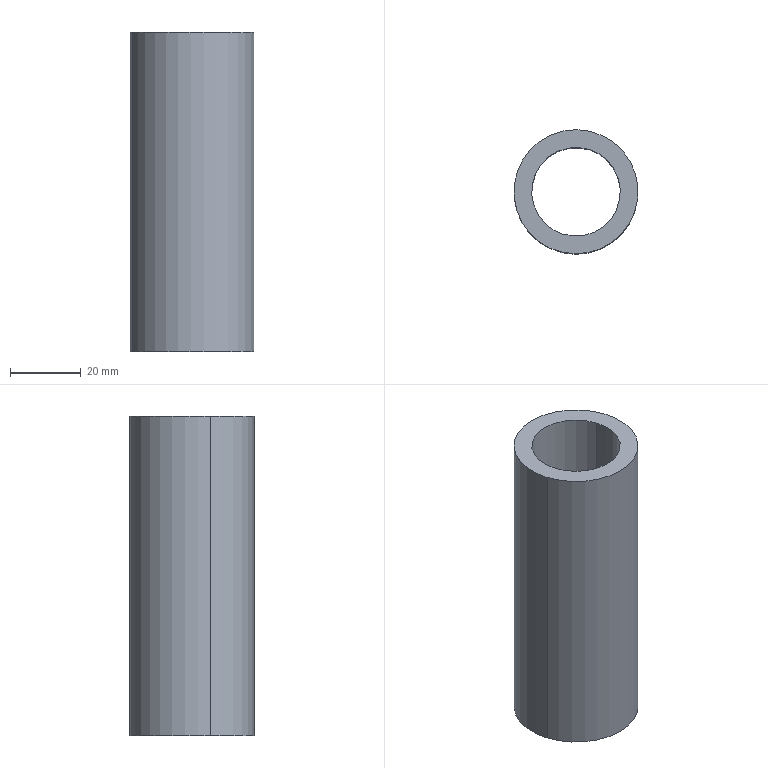Component | SolidWorks | UpperSideBeltXG-XG1-1_CopperSleeveXG-XG1-1 | 1 solid | 6 faces | box 35 x 35 x 90 mm | volume 42412 mm3 | cylinder 4 | plane 2 | commonest cylinder face diameters 25 x2 35 x2
build123d program:
from build123d import *

# Parameters (mm, degrees)
SKETCH1_R           = 17.5
SKETCH1_R_2         = 12.5
BOSS_EXTRUDE1_DEPTH = 90


with BuildPart() as part:
    # Sketch1 → Boss-Extrude1 (new body)
    with BuildSketch(Plane(origin=(0, 0, 0), x_dir=(1, 0, 0), z_dir=(0, 1, 0))):
        with Locations(Location((0, 0, 0), (0, 0, 90))):
            Circle(SKETCH1_R)
        with Locations(Location((0, 0, 0), (0, 0, 90))):
            Circle(SKETCH1_R_2, mode=Mode.SUBTRACT)
    extrude(amount=BOSS_EXTRUDE1_DEPTH)


solid = part.part

# Placed as in the assembly
solid = solid.moved(Location((-348.72, 395, 218), (90, 0, 0)))
STEP:
#1=CARTESIAN_POINT('',(-14.199,15.406,12.126));
#2=VERTEX_POINT('',#1);
#3=CARTESIAN_POINT('',(-13.259,15.697,12.126));
#4=VERTEX_POINT('',#3);
#5=CARTESIAN_POINT('',(-13.729,15.551,12.126));
#6=DIRECTION('',(0.,-0.,1.));
#7=DIRECTION('',(0.9554,0.2953,0.));
#8=AXIS2_PLACEMENT_3D('',#5,#6,#7);
#9=CIRCLE('',#8,0.4921);
#10=EDGE_CURVE('',#2,#4,#9,.T.);
#11=ORIENTED_EDGE('',*,*,#10,.T.);
#12=CARTESIAN_POINT('',(-13.259,15.697,8.583));
#13=VERTEX_POINT('',#12);
#14=CARTESIAN_POINT('',(-13.259,15.697,12.126));
#15=DIRECTION('',(-0.,0.,-1.));
#16=VECTOR('',#15,39.37);
#17=LINE('',#14,#16);
#18=EDGE_CURVE('',#4,#13,#17,.T.);
#19=ORIENTED_EDGE('',*,*,#18,.T.);
#20=CARTESIAN_POINT('',(-14.199,15.406,8.583));
#21=VERTEX_POINT('',#20);
#22=CARTESIAN_POINT('',(-13.729,15.551,8.583));
#23=DIRECTION('',(0.,-0.,1.));
#24=DIRECTION('',(0.9554,0.2953,0.));
#25=AXIS2_PLACEMENT_3D('',#22,#23,#24);
#26=CIRCLE('',#25,0.4921);
#27=EDGE_CURVE('',#21,#13,#26,.T.);
#28=ORIENTED_EDGE('',*,*,#27,.F.);
#29=CARTESIAN_POINT('',(-14.199,15.406,12.126));
#30=DIRECTION('',(-0.,0.,-1.));
#31=VECTOR('',#30,39.37);
#32=LINE('',#29,#31);
#33=EDGE_CURVE('',#2,#21,#32,.T.);
#34=ORIENTED_EDGE('',*,*,#33,.F.);
#35=EDGE_LOOP('',(#11,#19,#28,#34));
#36=FACE_OUTER_BOUND('',#35,.T.);
#37=CARTESIAN_POINT('',(-13.729,15.551,12.126));
#38=DIRECTION('',(-0.,0.,-1.));
#39=DIRECTION('',(-0.9554,-0.2953,0.));
#40=AXIS2_PLACEMENT_3D('',#37,#38,#39);
#41=CYLINDRICAL_SURFACE('',#40,0.4921);
#42=ADVANCED_FACE('',(#36),#41,.F.);
#43=CARTESIAN_POINT('',(-13.071,15.755,12.126));
#44=VERTEX_POINT('',#43);
#45=CARTESIAN_POINT('',(-14.387,15.348,12.126));
#46=VERTEX_POINT('',#45);
#47=CARTESIAN_POINT('',(-13.729,15.551,12.126));
#48=DIRECTION('',(0.,-0.,1.));
#49=DIRECTION('',(0.9554,0.2953,0.));
#50=AXIS2_PLACEMENT_3D('',#47,#48,#49);
#51=CIRCLE('',#50,0.689);
#52=EDGE_CURVE('',#44,#46,#51,.T.);
#53=ORIENTED_EDGE('',*,*,#52,.F.);
#54=CARTESIAN_POINT('',(-13.071,15.755,8.583));
#55=VERTEX_POINT('',#54);
#56=CARTESIAN_POINT('',(-13.071,15.755,12.126));
#57=DIRECTION('',(-0.,0.,-1.));
#58=VECTOR('',#57,39.37);
#59=LINE('',#56,#58);
#60=EDGE_CURVE('',#44,#55,#59,.T.);
#61=ORIENTED_EDGE('',*,*,#60,.T.);
#62=CARTESIAN_POINT('',(-14.387,15.348,8.583));
#63=VERTEX_POINT('',#62);
#64=CARTESIAN_POINT('',(-13.729,15.551,8.583));
#65=DIRECTION('',(0.,-0.,1.));
#66=DIRECTION('',(0.9554,0.2953,0.));
#67=AXIS2_PLACEMENT_3D('',#64,#65,#66);
#68=CIRCLE('',#67,0.689);
#69=EDGE_CURVE('',#55,#63,#68,.T.);
#70=ORIENTED_EDGE('',*,*,#69,.T.);
#71=CARTESIAN_POINT('',(-14.387,15.348,12.126));
#72=DIRECTION('',(-0.,0.,-1.));
#73=VECTOR('',#72,39.37);
#74=LINE('',#71,#73);
#75=EDGE_CURVE('',#46,#63,#74,.T.);
#76=ORIENTED_EDGE('',*,*,#75,.F.);
#77=EDGE_LOOP('',(#53,#61,#70,#76));
#78=FACE_OUTER_BOUND('',#77,.T.);
#79=CARTESIAN_POINT('',(-13.729,15.551,12.126));
#80=DIRECTION('',(-0.,0.,-1.));
#81=DIRECTION('',(-0.9554,-0.2953,0.));
#82=AXIS2_PLACEMENT_3D('',#79,#80,#81);
#83=CYLINDRICAL_SURFACE('',#82,0.689);
#84=ADVANCED_FACE('',(#78),#83,.T.);
#85=CARTESIAN_POINT('',(-13.729,15.551,12.126));
#86=DIRECTION('',(0.,-0.,1.));
#87=DIRECTION('',(0.9554,0.2953,0.));
#88=AXIS2_PLACEMENT_3D('',#85,#86,#87);
#89=CIRCLE('',#88,0.689);
#90=EDGE_CURVE('',#46,#44,#89,.T.);
#91=ORIENTED_EDGE('',*,*,#90,.T.);
#92=ORIENTED_EDGE('',*,*,#52,.T.);
#93=EDGE_LOOP('',(#91,#92));
#94=FACE_OUTER_BOUND('',#93,.T.);
#95=ORIENTED_EDGE('',*,*,#10,.F.);
#96=CARTESIAN_POINT('',(-13.729,15.551,12.126));
#97=DIRECTION('',(0.,-0.,1.));
#98=DIRECTION('',(0.9554,0.2953,0.));
#99=AXIS2_PLACEMENT_3D('',#96,#97,#98);
#100=CIRCLE('',#99,0.4921);
#101=EDGE_CURVE('',#4,#2,#100,.T.);
#102=ORIENTED_EDGE('',*,*,#101,.F.);
#103=EDGE_LOOP('',(#95,#102));
#104=FACE_BOUND('',#103,.T.);
#105=CARTESIAN_POINT('',(-13.729,15.551,12.126));
#106=DIRECTION('',(0.,-0.,1.));
#107=DIRECTION('',(0.9554,0.2953,-0.));
#108=AXIS2_PLACEMENT_3D('',#105,#106,#107);
#109=PLANE('',#108);
#110=ADVANCED_FACE('',(#94,#104),#109,.T.);
#111=CARTESIAN_POINT('',(-13.729,15.551,8.583));
#112=DIRECTION('',(0.,-0.,1.));
#113=DIRECTION('',(0.9554,0.2953,0.));
#114=AXIS2_PLACEMENT_3D('',#111,#112,#113);
#115=CIRCLE('',#114,0.689);
#116=EDGE_CURVE('',#63,#55,#115,.T.);
#117=ORIENTED_EDGE('',*,*,#116,.F.);
#118=ORIENTED_EDGE('',*,*,#69,.F.);
#119=EDGE_LOOP('',(#117,#118));
#120=FACE_OUTER_BOUND('',#119,.T.);
#121=ORIENTED_EDGE('',*,*,#27,.T.);
#122=CARTESIAN_POINT('',(-13.729,15.551,8.583));
#123=DIRECTION('',(0.,-0.,1.));
#124=DIRECTION('',(0.9554,0.2953,0.));
#125=AXIS2_PLACEMENT_3D('',#122,#123,#124);
#126=CIRCLE('',#125,0.4921);
#127=EDGE_CURVE('',#13,#21,#126,.T.);
#128=ORIENTED_EDGE('',*,*,#127,.T.);
#129=EDGE_LOOP('',(#121,#128));
#130=FACE_BOUND('',#129,.T.);
#131=CARTESIAN_POINT('',(-13.729,15.551,8.583));
#132=DIRECTION('',(0.,-0.,1.));
#133=DIRECTION('',(0.9554,0.2953,-0.));
#134=AXIS2_PLACEMENT_3D('',#131,#132,#133);
#135=PLANE('',#134);
#136=ADVANCED_FACE('',(#120,#130),#135,.F.);
#137=ORIENTED_EDGE('',*,*,#60,.F.);
#138=ORIENTED_EDGE('',*,*,#90,.F.);
#139=ORIENTED_EDGE('',*,*,#75,.T.);
#140=ORIENTED_EDGE('',*,*,#116,.T.);
#141=EDGE_LOOP('',(#137,#138,#139,#140));
#142=FACE_OUTER_BOUND('',#141,.T.);
#143=CARTESIAN_POINT('',(-13.729,15.551,12.126));
#144=DIRECTION('',(-0.,0.,-1.));
#145=DIRECTION('',(-0.9554,-0.2953,0.));
#146=AXIS2_PLACEMENT_3D('',#143,#144,#145);
#147=CYLINDRICAL_SURFACE('',#146,0.689);
#148=ADVANCED_FACE('',(#142),#147,.T.);
#149=ORIENTED_EDGE('',*,*,#18,.F.);
#150=ORIENTED_EDGE('',*,*,#101,.T.);
#151=ORIENTED_EDGE('',*,*,#33,.T.);
#152=ORIENTED_EDGE('',*,*,#127,.F.);
#153=EDGE_LOOP('',(#149,#150,#151,#152));
#154=FACE_OUTER_BOUND('',#153,.T.);
#155=CARTESIAN_POINT('',(-13.729,15.551,12.126));
#156=DIRECTION('',(-0.,0.,-1.));
#157=DIRECTION('',(-0.9554,-0.2953,0.));
#158=AXIS2_PLACEMENT_3D('',#155,#156,#157);
#159=CYLINDRICAL_SURFACE('',#158,0.4921);
#160=ADVANCED_FACE('',(#154),#159,.F.);
#161=CLOSED_SHELL('',(#42,#84,#110,#136,#148,#160));
#162=MANIFOLD_SOLID_BREP('',#161);
#163=CARTESIAN_POINT('',(0.,0.,0.));
#164=DIRECTION('',(0.,0.,1.));
#165=DIRECTION('',(1.,0.,0.));
#166=AXIS2_PLACEMENT_3D('',#163,#164,#165);
#167=(LENGTH_UNIT()NAMED_UNIT(*)SI_UNIT($,.METRE.));
#168=LENGTH_MEASURE_WITH_UNIT(LENGTH_MEASURE(0.0254),#167);
#169=DIMENSIONAL_EXPONENTS(1.,0.,0.,0.,0.,0.,0.);
#170=(CONVERSION_BASED_UNIT('',#168)LENGTH_UNIT()NAMED_UNIT(#169));
#171=UNCERTAINTY_MEASURE_WITH_UNIT(LENGTH_MEASURE(0.00001),#170,'','');
#172=(NAMED_UNIT(*)PLANE_ANGLE_UNIT()SI_UNIT($,.RADIAN.));
#173=(NAMED_UNIT(*)SI_UNIT($,.STERADIAN.)SOLID_ANGLE_UNIT());
#174=(GEOMETRIC_REPRESENTATION_CONTEXT(3)GLOBAL_UNCERTAINTY_ASSIGNED_CONTEXT((#171))GLOBAL_UNIT_ASSIGNED_CONTEXT((#170,#172,#173))REPRESENTATION_CONTEXT('',''));
#175=ADVANCED_BREP_SHAPE_REPRESENTATION('',(#162,#166),#174);
#176=COLOUR_RGB('',0.7922,0.8196,0.9333);
#177=FILL_AREA_STYLE_COLOUR('',#176);
#178=FILL_AREA_STYLE('',(#177));
#179=SURFACE_STYLE_FILL_AREA(#178);
#180=SURFACE_SIDE_STYLE('',(#179));
#181=SURFACE_STYLE_USAGE(.BOTH.,#180);
#182=PRESENTATION_STYLE_ASSIGNMENT((#181));
#183=STYLED_ITEM('',(#182),#162);
#184=(LENGTH_UNIT()NAMED_UNIT(*)SI_UNIT($,.METRE.));
#185=LENGTH_MEASURE_WITH_UNIT(LENGTH_MEASURE(0.0254),#184);
#186=DIMENSIONAL_EXPONENTS(1.,0.,0.,0.,0.,0.,0.);
#187=(CONVERSION_BASED_UNIT('',#185)LENGTH_UNIT()NAMED_UNIT(#186));
#188=UNCERTAINTY_MEASURE_WITH_UNIT(LENGTH_MEASURE(0.00001),#187,'','');
#189=(NAMED_UNIT(*)PLANE_ANGLE_UNIT()SI_UNIT($,.RADIAN.));
#190=(NAMED_UNIT(*)SI_UNIT($,.STERADIAN.)SOLID_ANGLE_UNIT());
#191=(GEOMETRIC_REPRESENTATION_CONTEXT(3)GLOBAL_UNCERTAINTY_ASSIGNED_CONTEXT((#188))GLOBAL_UNIT_ASSIGNED_CONTEXT((#187,#189,#190))REPRESENTATION_CONTEXT('',''));
#192=MECHANICAL_DESIGN_GEOMETRIC_PRESENTATION_REPRESENTATION('',(#183),#191);
#193=PRESENTATION_LAYER_ASSIGNMENT('','',(#183));